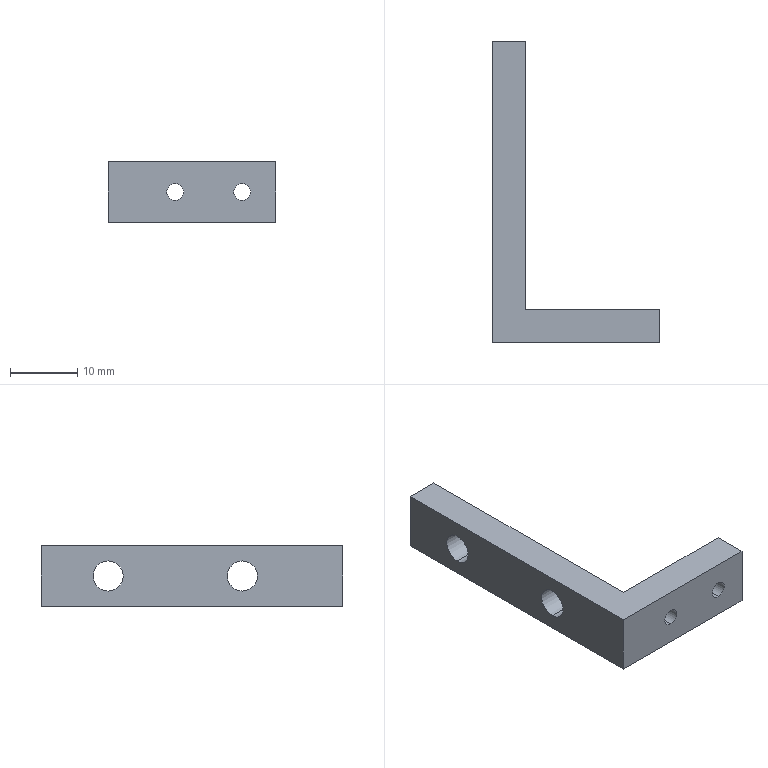CAM job | Mastercam | mm | 10 operations | part box 25 x 45 x 9
1. Facing | 20 - 63 平铣刀
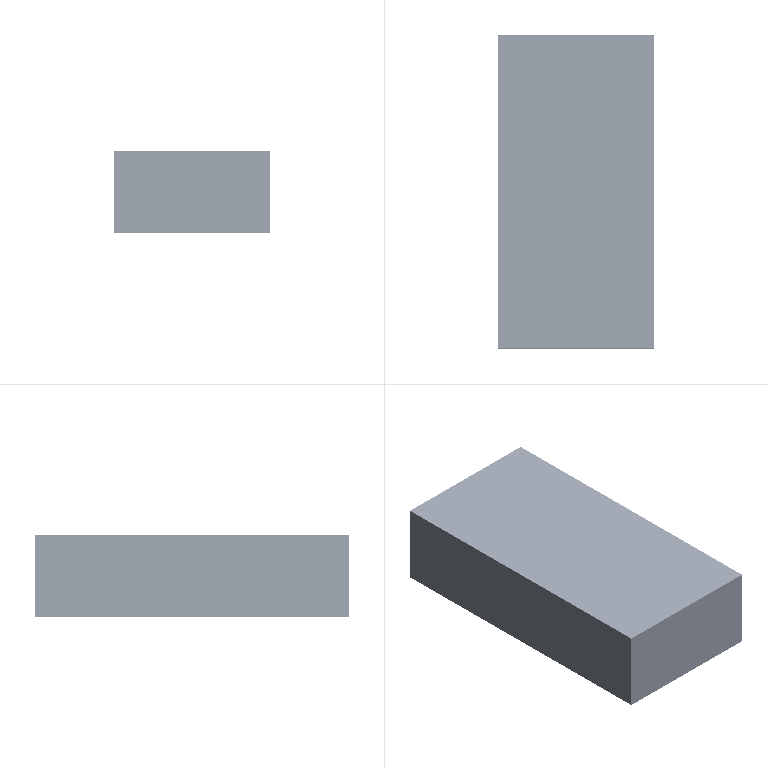2. Contour (Ramp) | 12 - 12 平铣刀
3. Contour (2D) | 12 - 12 平铣刀
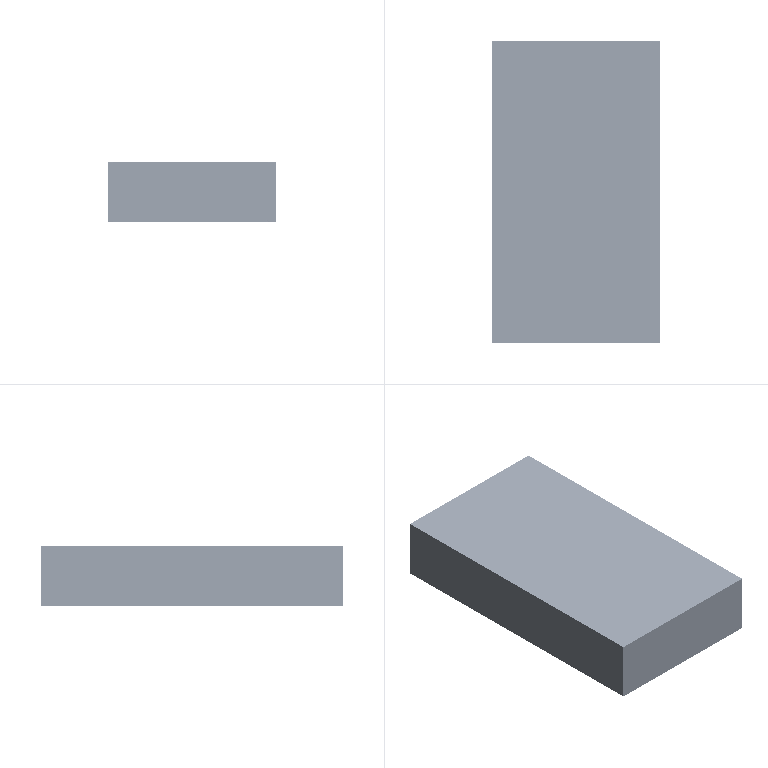4. Contour (2D chamfer) | 7 - 4 倒角刀
5. Facing | 20 - 63 平铣刀
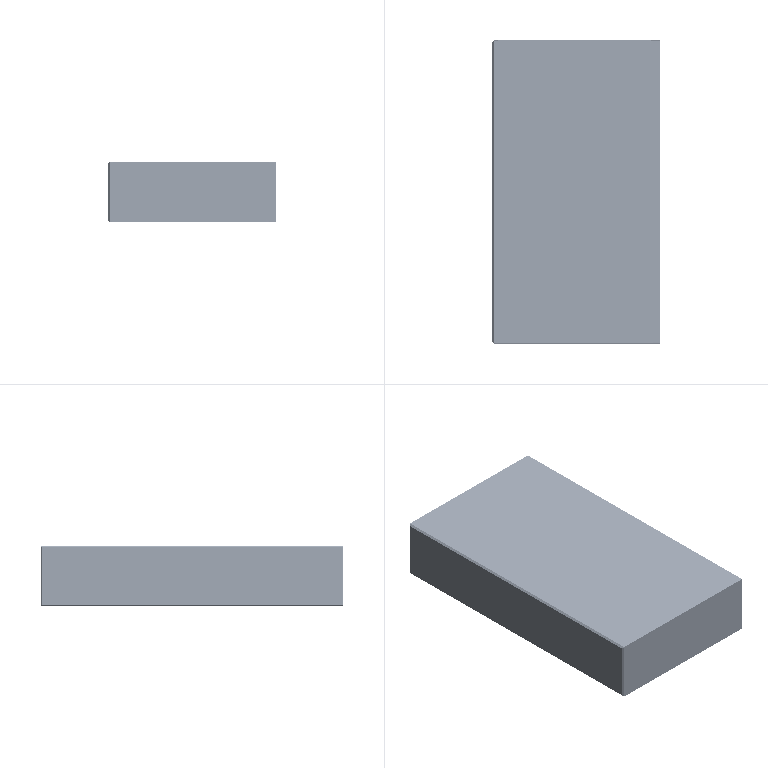6. Contour (2D chamfer) | 7 - 4 倒角刀
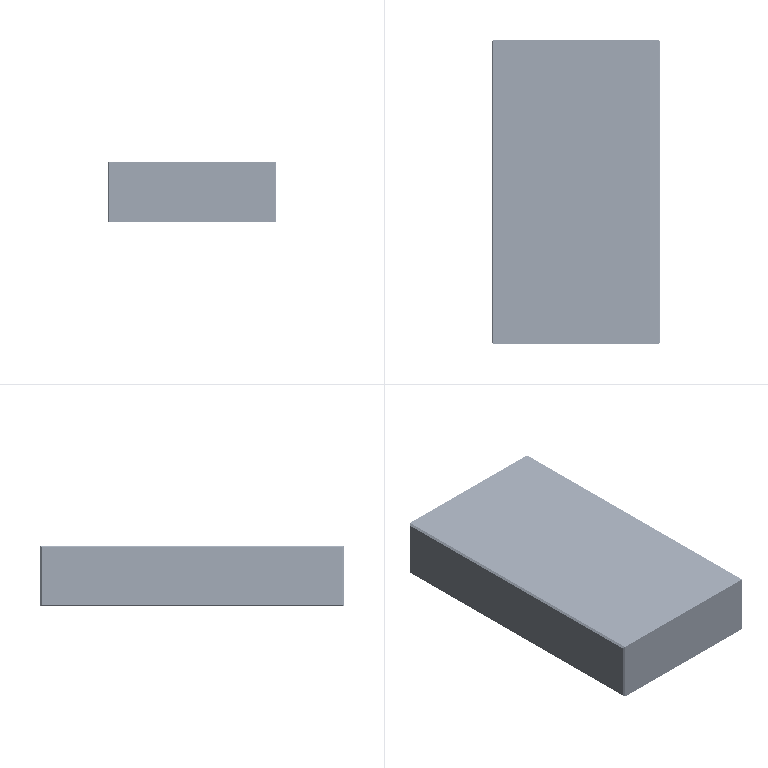7. Drill/Counterbore | 7 - 4 倒角刀
8. Contour (Ramp) | 12 - 12 平铣刀
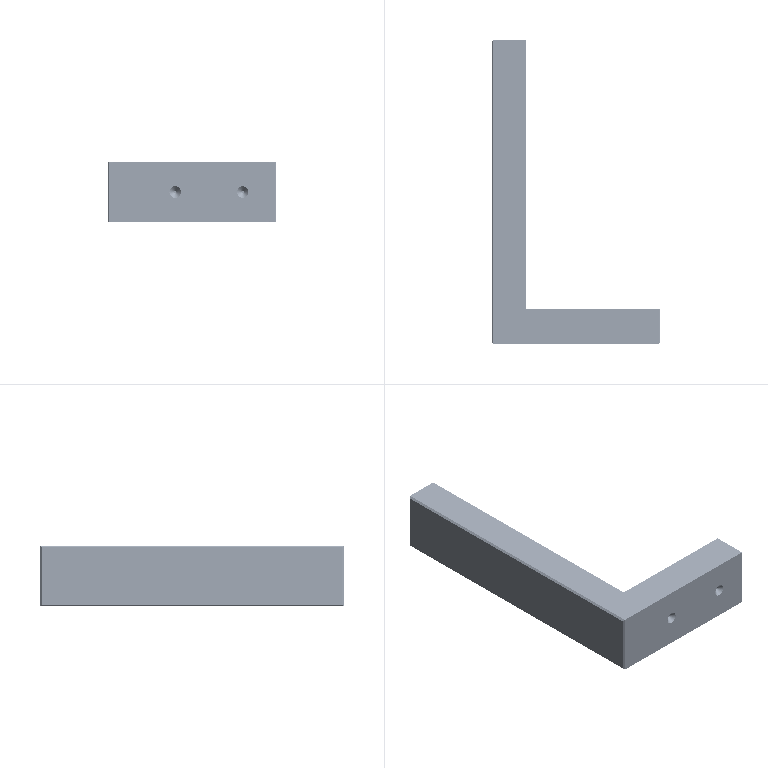9. Contour (2D) | 12 - 12 平铣刀
10. Drill/Counterbore | 7 - 4 倒角刀